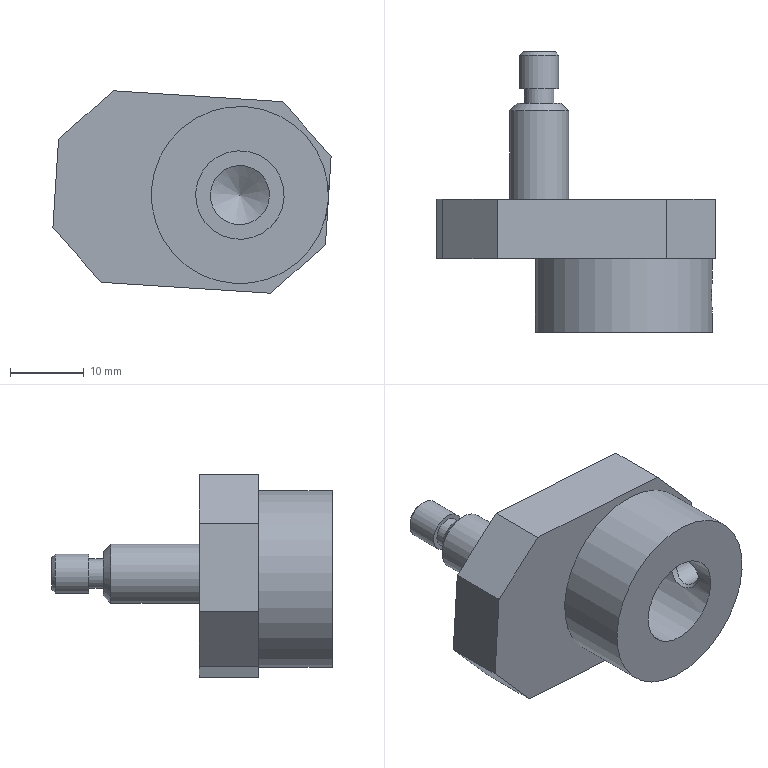Component | NX | CLHKJG_13_ECCENTRIC_SLEEVE | 1 solid | 27 faces | volume 10577 mm3 | plane 15 | cylinder 7 | cone 3 | spline 2 | commonest cylinder face diameters 8 x2 24 x1 4 x1 5.304 x1 12 x1 4.2 x1